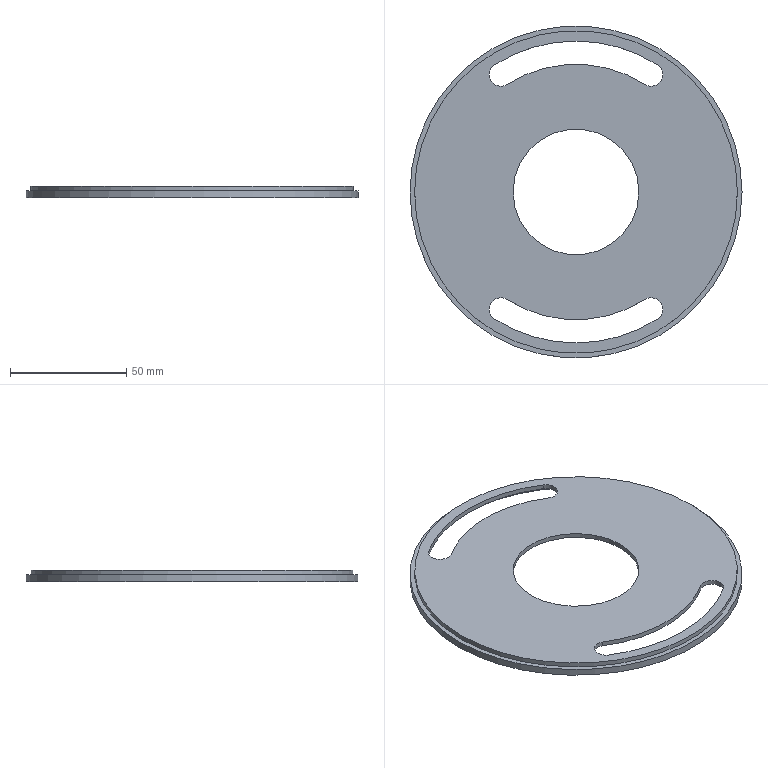Component | NX | BAFFLE | 1 solid | 16 faces | volume 26648 mm3 | cylinder 12 | plane 4 | commonest cylinder face diameters 10.023 x4 130 x2 110 x2 54.2 x1 139 x1 143 x1 137 x1